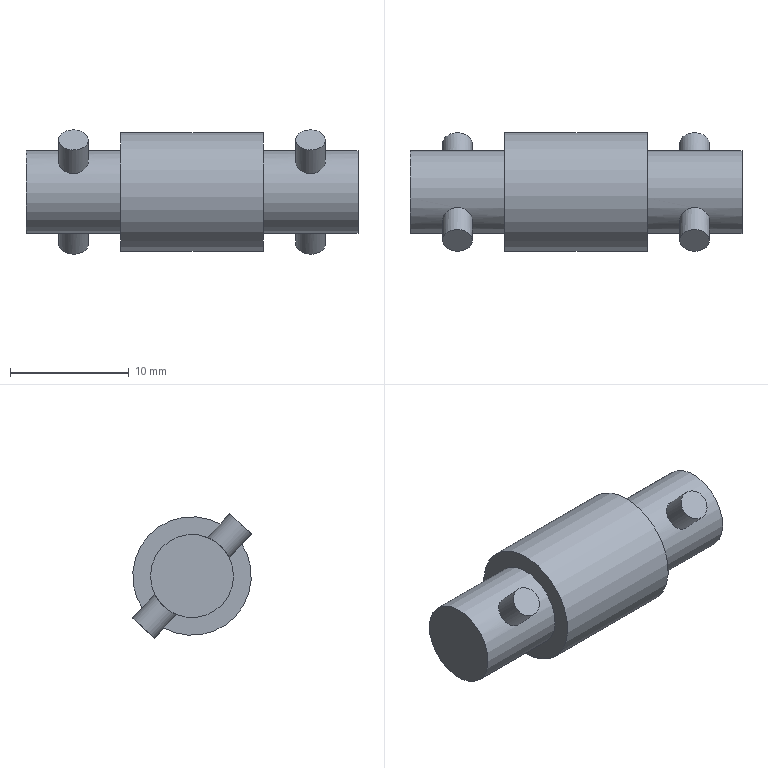Component | NX | 15D__27 | 1 solid | 15 faces | volume 1608 mm3 | plane 8 | cylinder 7 | commonest cylinder face diameters 2.5 x4 7 x2 10 x1